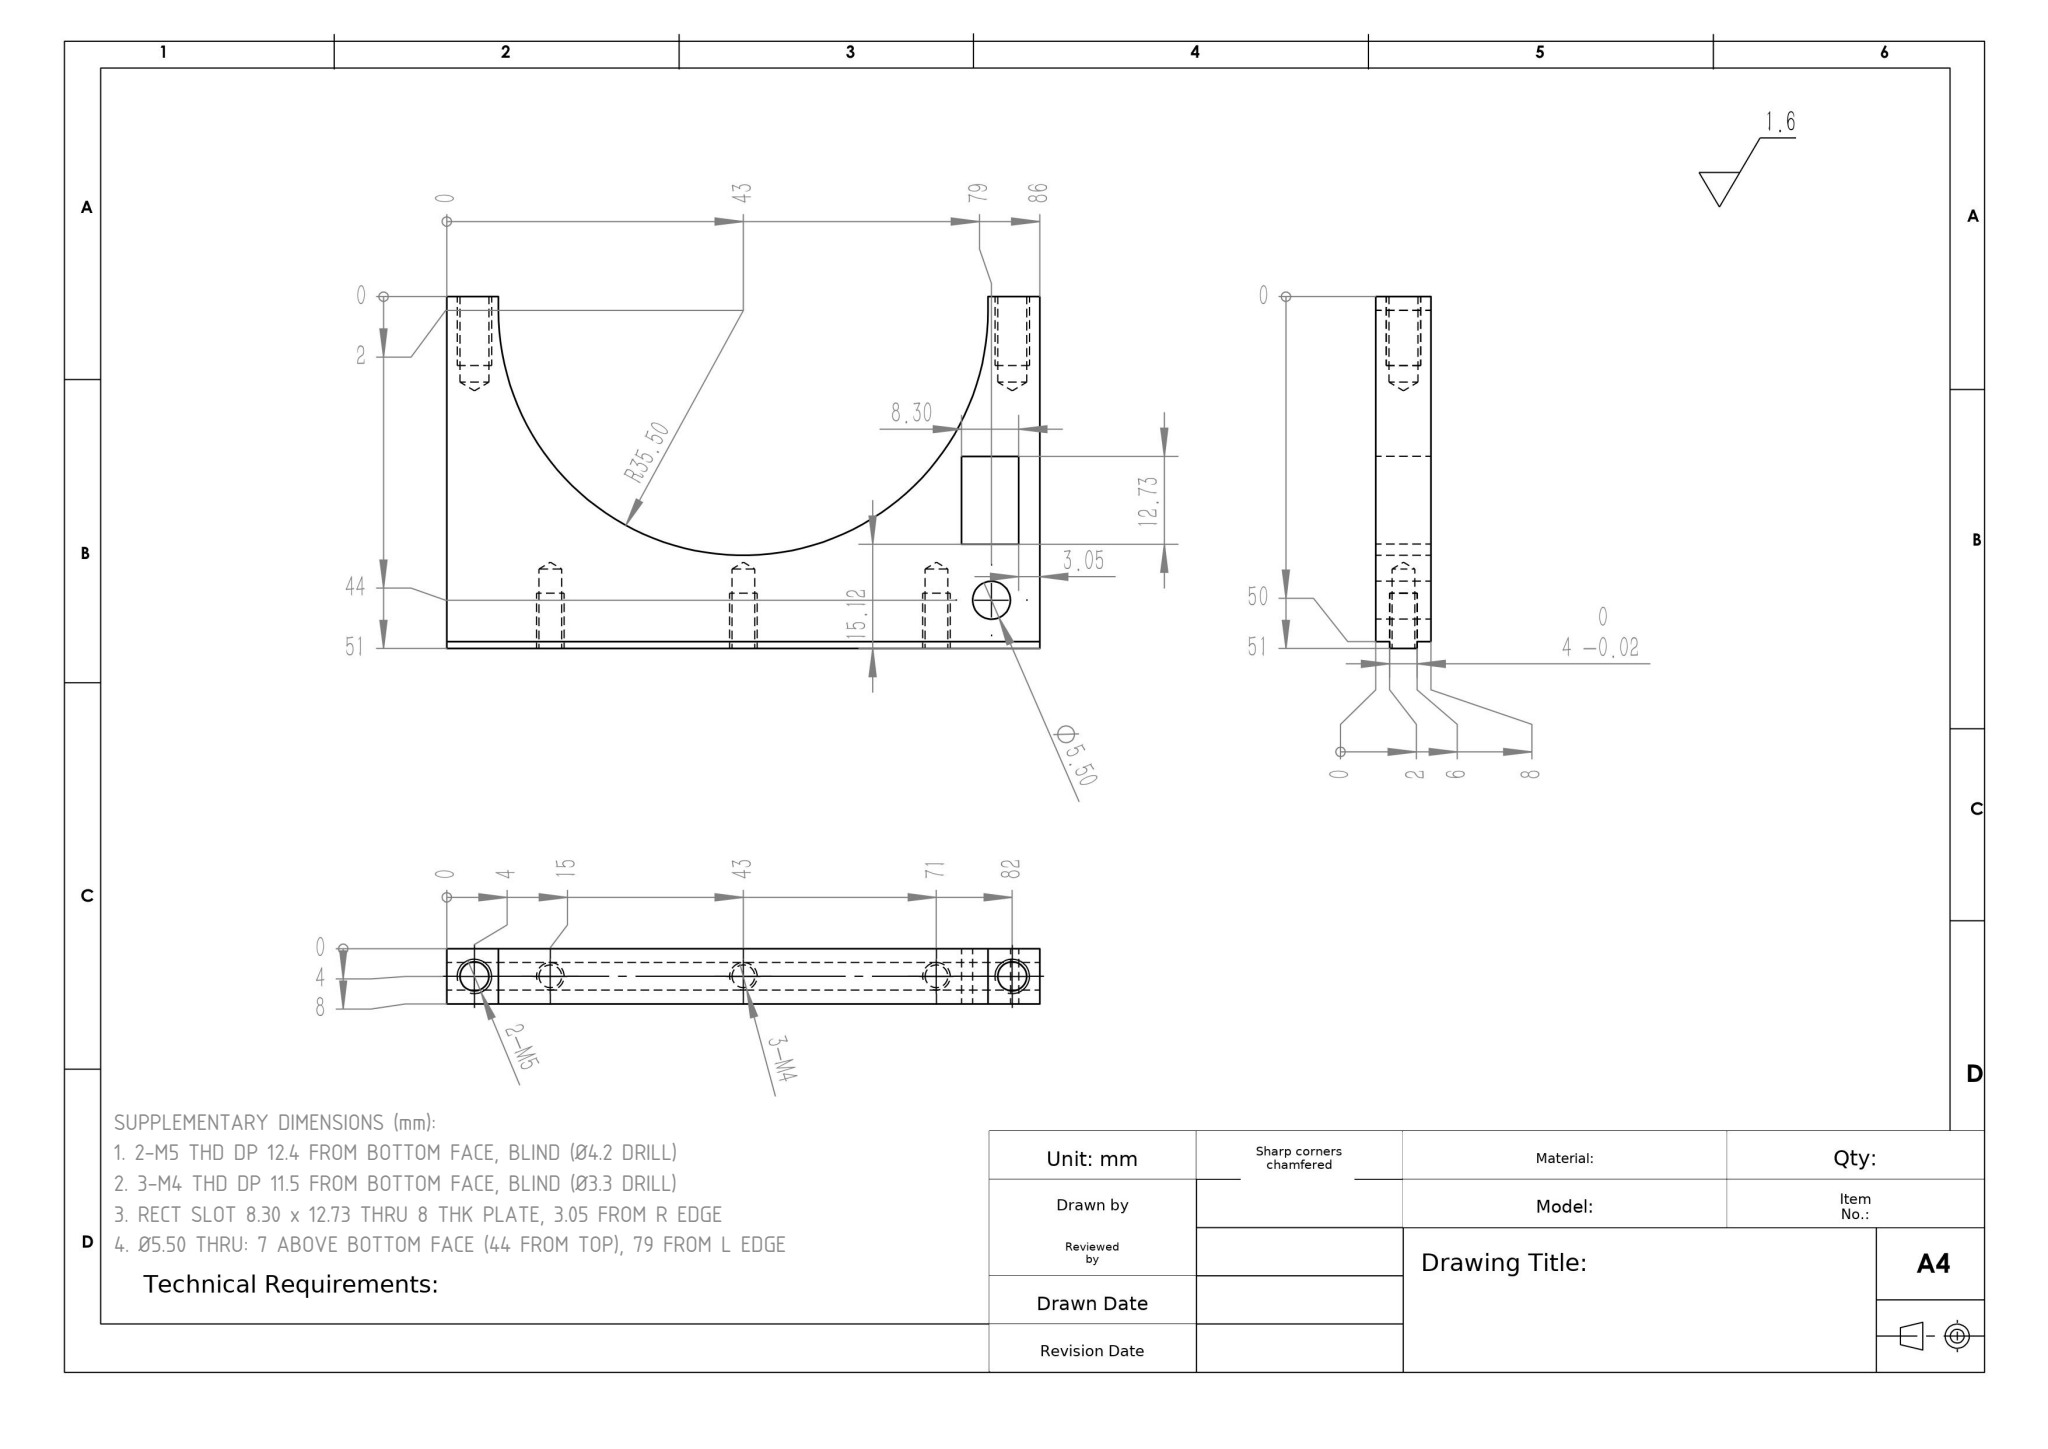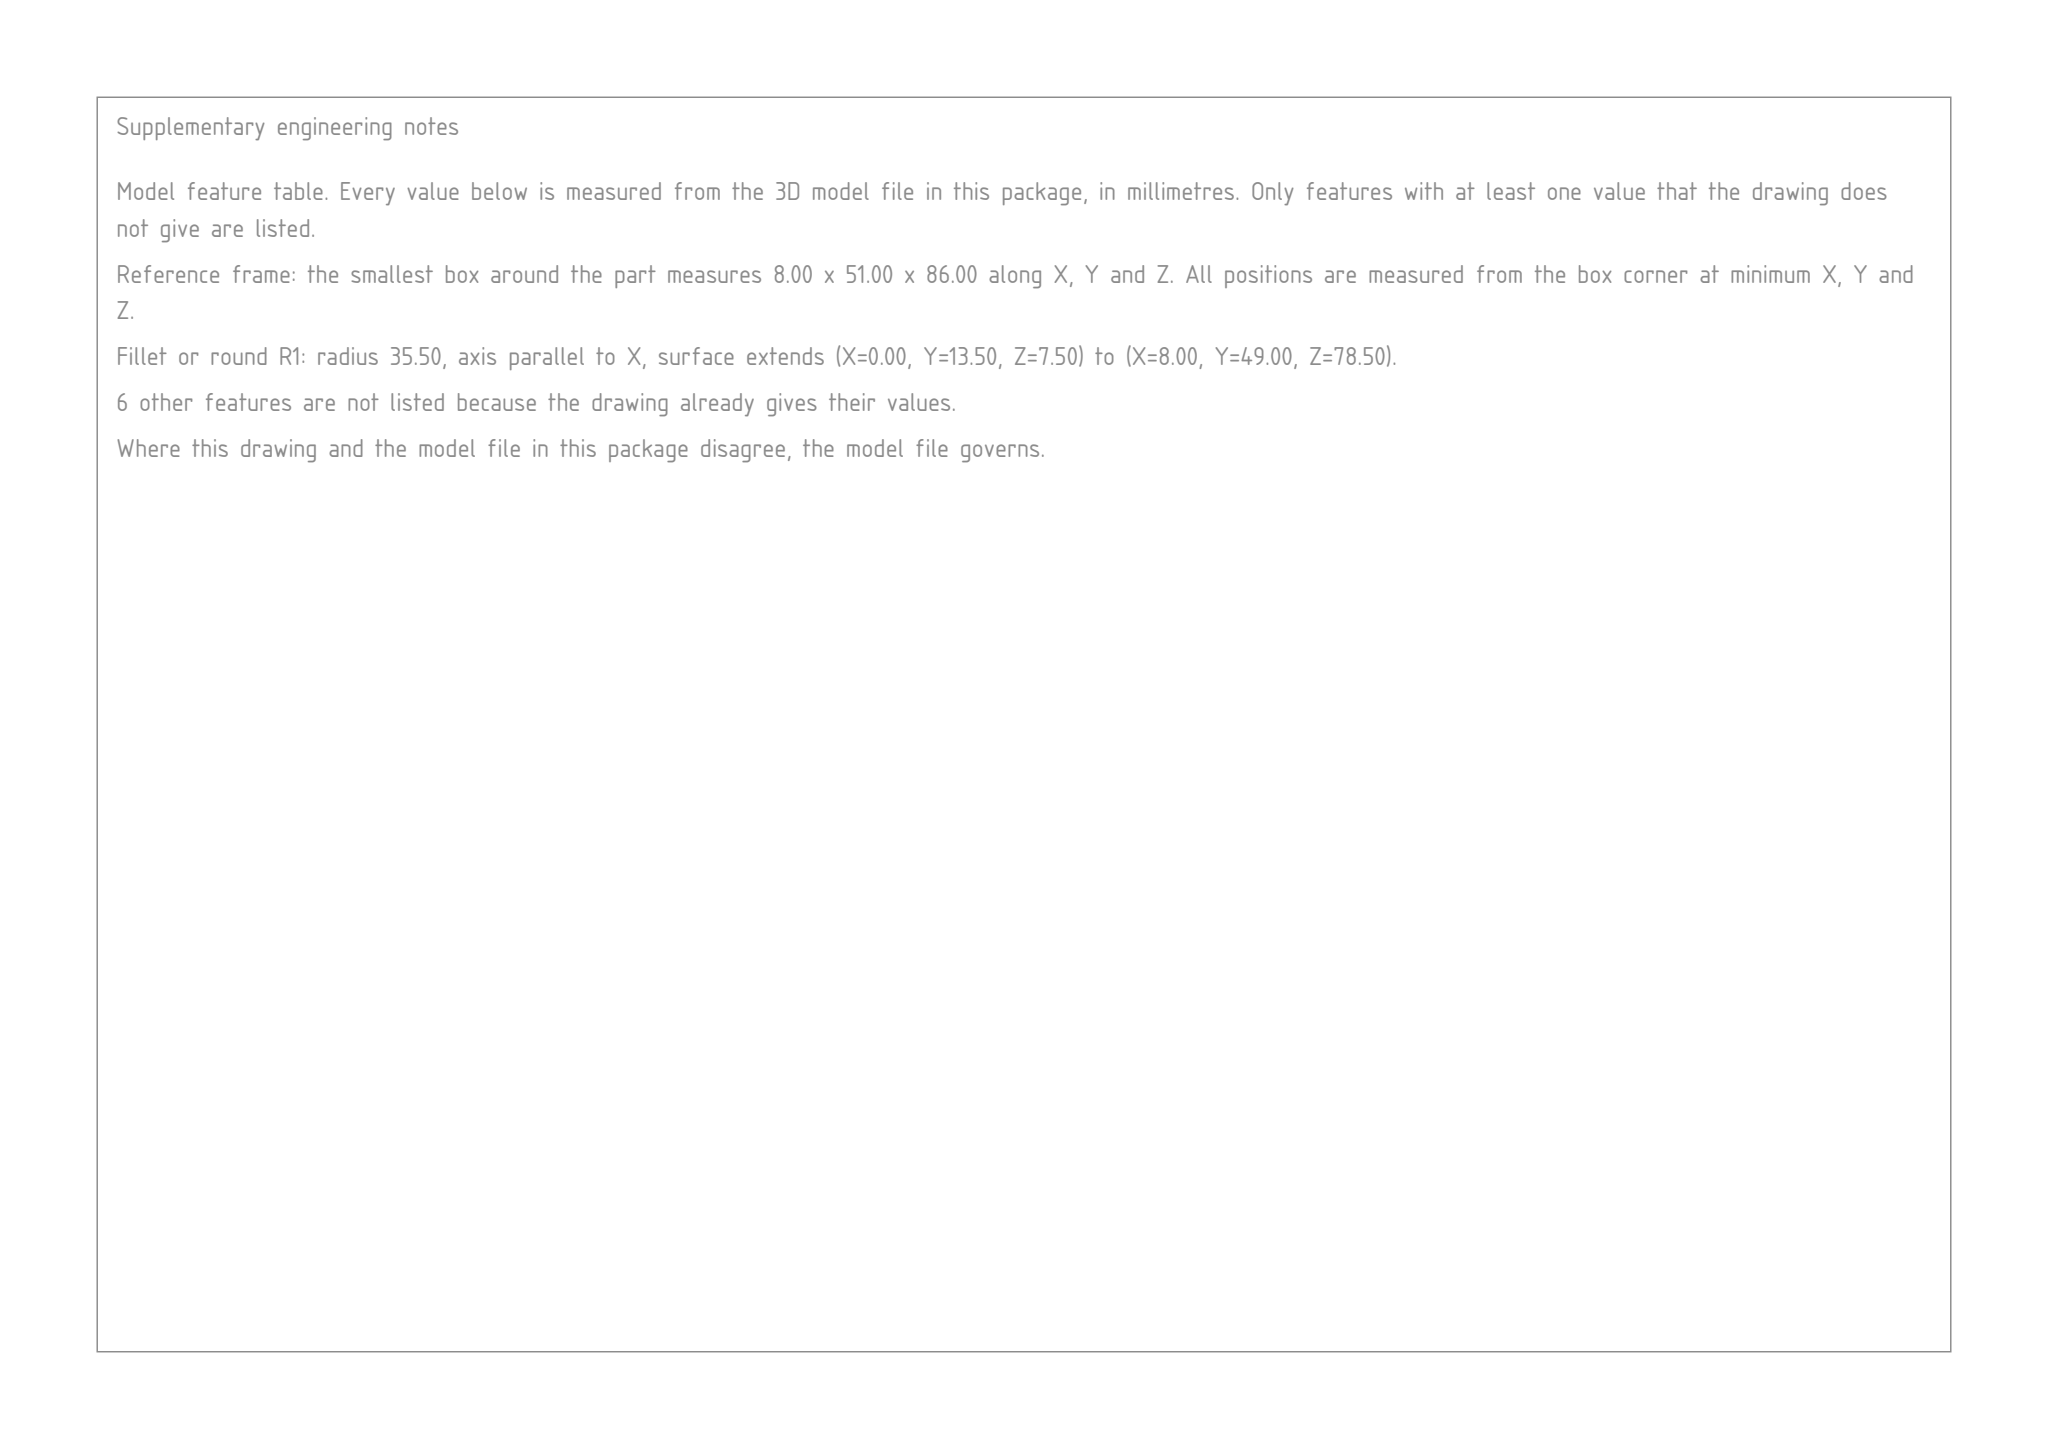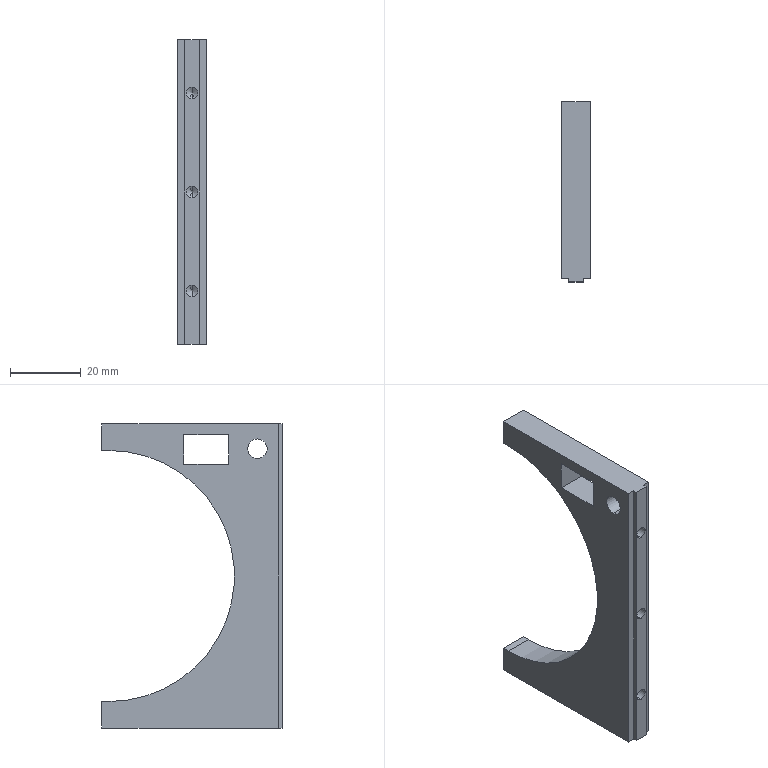Part | SolidWorks | mm | 1 solid | 40 faces | box 8 x 51 x 86 mm | volume 16077 mm3 | plane 17 | cylinder 13 | cone 10 | commonest cylinder face diameters 3.3 x6 4.2 x4 5.5 x2 71 x1
build123d program:
from build123d import *

# Parameters (mm, degrees)
SKETCH1_W                      = 8
SKETCH1_H                      = 50
BOSS_EXTRUDE1_DEPTH            = 86
CUT_EXTRUDE1_DEPTH             = 100.8
SKETCH7_W                      = 4
SKETCH7_H                      = 1
BOSS_EXTRUDE2_DEPTH            = 86
F_5_5_5_5_DIAMETER_HOLE1_D     = 5.5
F_5_5_5_5_DIAMETER_HOLE1_DEPTH = 10
F_5_5_5_5_DIAMETER_HOLE1_TIP   = 1.652
M5_TAPPED_HOLE1_D              = 4.2
M5_TAPPED_HOLE1_DEPTH          = 12.4
M5_TAPPED_HOLE1_TIP            = 1.262
M4_TAPPED_HOLE1_D              = 3.3
M4_TAPPED_HOLE1_DEPTH          = 11.5
M4_TAPPED_HOLE1_TIP            = 0.9914
SKETCH12_W                     = 8.302
SKETCH12_H                     = 12.725
CUT_EXTRUDE2_DEPTH             = 28


with BuildPart() as part:
    # Sketch1 → Boss-Extrude1 (new body)
    with BuildSketch(Plane.XY):
        with Locations((4, 25)):
            Rectangle(SKETCH1_W, SKETCH1_H)
    extrude(amount=BOSS_EXTRUDE1_DEPTH)

    # Sketch2 → Cut-Extrude1 (cut, through all)
    with BuildSketch(Plane(origin=(8, 0, 0), x_dir=(0, 0, -1), z_dir=(1, 0, 0))):
        with BuildLine():
            Line((-7.5, 48), (-7.5, 76))
            Line((-7.5, 76), (-78.5, 76))
            Line((-78.5, 76), (-78.5, 48))
            ThreePointArc((-78.5, 48), (-43, 12.5), (-7.5, 48))
        make_face()
    extrude(amount=-CUT_EXTRUDE1_DEPTH, mode=Mode.SUBTRACT)

    # Sketch7 → Boss-Extrude2 (add)
    with BuildSketch(Plane(origin=(0, 0, 0), x_dir=(-1, 0, 0), z_dir=(0, 0, -1))):
        with Locations((-4, -0.5)):
            Rectangle(SKETCH7_W, SKETCH7_H)
    extrude(amount=-BOSS_EXTRUDE2_DEPTH)

    # 5.5 _5.5_ Diameter Hole1
    with Locations(Plane(origin=(0, 6, 79), x_dir=(0, 0, -1), z_dir=(-1, 0, 0))):
        with Locations((0, 0)):
            Hole(F_5_5_5_5_DIAMETER_HOLE1_D / 2, depth=F_5_5_5_5_DIAMETER_HOLE1_DEPTH)
            with Locations((0, 0, -(F_5_5_5_5_DIAMETER_HOLE1_DEPTH + F_5_5_5_5_DIAMETER_HOLE1_TIP / 2))):  # 118° drill point
                Cone(0, F_5_5_5_5_DIAMETER_HOLE1_D / 2, F_5_5_5_5_DIAMETER_HOLE1_TIP, mode=Mode.SUBTRACT)

    # M5 Tapped Hole1
    with Locations(Plane(origin=(4, 50, 82), x_dir=(0, 0, 1), z_dir=(0, 1, 0))):
        with Locations((0, 0), (-78, 0)):
            Hole(M5_TAPPED_HOLE1_D / 2, depth=M5_TAPPED_HOLE1_DEPTH)
            with Locations((0, 0, -(M5_TAPPED_HOLE1_DEPTH + M5_TAPPED_HOLE1_TIP / 2))):  # 118° drill point
                Cone(0, M5_TAPPED_HOLE1_D / 2, M5_TAPPED_HOLE1_TIP, mode=Mode.SUBTRACT)

    # M4 Tapped Hole1
    with Locations(Plane(origin=(4, -1, 71), x_dir=(-1, 0, 0), z_dir=(0, -1, 0))):
        with Locations((0, 0), (0, 28), (0, 56)):
            Hole(M4_TAPPED_HOLE1_D / 2, depth=M4_TAPPED_HOLE1_DEPTH)
            with Locations((0, 0, -(M4_TAPPED_HOLE1_DEPTH + M4_TAPPED_HOLE1_TIP / 2))):  # 118° drill point
                Cone(0, M4_TAPPED_HOLE1_D / 2, M4_TAPPED_HOLE1_TIP, mode=Mode.SUBTRACT)

    # Sketch12 → Cut-Extrude2 (cut)
    with BuildSketch(Plane(origin=(8, 0, 0), x_dir=(0, 0, -1), z_dir=(1, 0, 0))):
        with Locations((-78.794, 20.485)):
            Rectangle(SKETCH12_W, SKETCH12_H)
    extrude(amount=-CUT_EXTRUDE2_DEPTH, mode=Mode.SUBTRACT)


solid = part.part